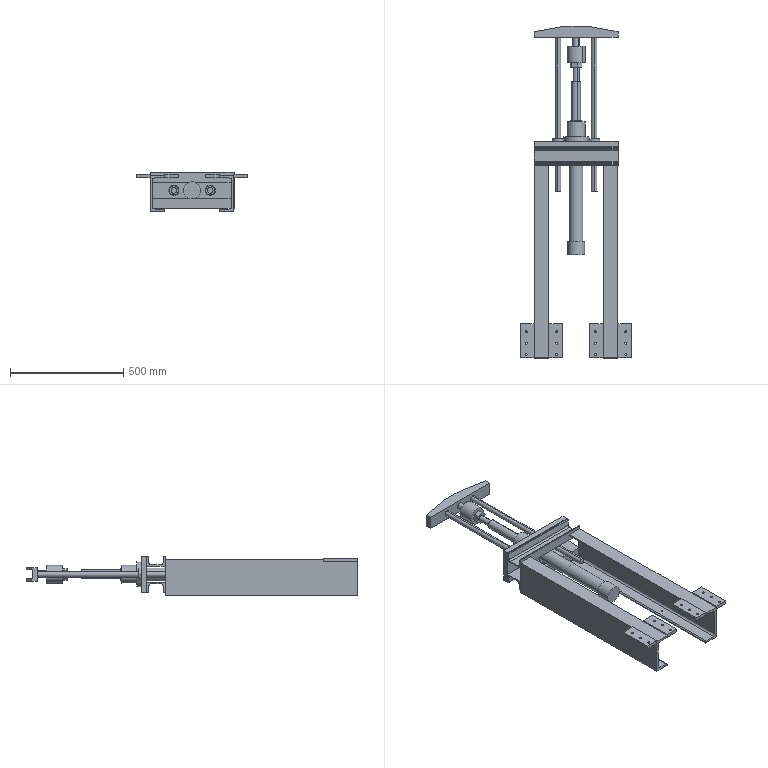Assembly | SolidWorks | mm | 17 component files | 17 solids | 221 faces | box 489.4 x 1462.46 x 173.22 mm | volume 10389265 mm3 | plane 115 | cylinder 98 | cone 8 | commonest cylinder face diameters 8.5 x16 10 x12 25 x12 40 x8 50 x8 5 x4 20 x4 60 x4
Bill of materials:
15mmSteelPlate2-331MachineTool | 2 |  | Flat rectangular plate with three round through holes in a row along its long axis; the middle hole is larger than the two end holes.
15mmSteelPlate-331MachineTool | 2 |  | Flat rectangular plate with three round through holes in a row along its length; the middle hole is larger.
BalanceCylinderBody | 1 |  | Long, slender, solid round shaft that is stepped along its axis. It has an enlarged cylindrical end section at one end, a thin raised collar near the other end, a short larger-diameter section beyond the collar, and a small step at that end's tip.
BalanceCylinderLever | 1 |  | Long, slender, solid stepped round pin: a short larger-diameter section at one end, a long middle shank, and a short reduced-diameter tip at the other end.
ChannelSteelNo.8470-2-650-331Machine | 1 |  | Short channel-section piece shown with the open side facing down (inverted U). It has one round through hole in the center of the web. The flanges taper and have rounded inner root fillets and rounded tips.
ChannelSteelNo.8470-650-331Machine | 1 |  | Straight length of channel section shown with the open side up. It has tapered flanges, rounded inner root fillets and rounded flange tips, and no holes are visible.
FloatingJointJA140-30-150 | 1 |  | Turned stepped part with a large cylindrical main body. One end has a smaller hexagonal boss with a central bore; the other end has a smaller solid cylindrical pin, coaxial with the body.
GuideRod-331 | 2 |  | Plain straight solid cylindrical rod of constant diameter with flat ends.
LinearBearingSchematic | 2 |  | Long channel section with the web vertical and the flanges pointing to one side (C-shape). The flanges taper and have rounded root fillets and tips. There is a very small dot-like mark on one flange.
NitrogenSupportChannelSteel65016a-2-331MachineTool | 1 |  | Long channel section (C-shape) with tapered flanges, rounded root fillets and rounded flange tips. No holes or other features are visible.
NitrogenSupportChannelSteel65016a-331MachineTool | 1 |  | Thin flat rectangular plate with three round through holes centered in a row along its length; the middle hole is larger than the two outer holes.
NitrogenSupportUpperPlate-331MachineTool | 1 |  | Flanged cylindrical sleeve: a hollow cylinder with a concentric through bore and a larger-diameter flange at one end.
SupportPlate-331 | 1 |  | Elongated straight bar with a C-shaped (channel-like) cross-section. Three round through holes in a row pass through the flat web: a larger hole in the middle and two smaller holes of equal size placed symmetrically on either side. Viewed from the side, the profile is symmetric: a flat raised middle section with straight tapers down toward both ends, so the flanges stand out farthest at mid-length and least at the ends.
Mates:
1. coincident | NitrogenSupportChannelSteel65016a-331MachineTool-1 face at (64.219, -126.562, 611.875) dir (0, -1, 0) | 15mmSteelPlate-331MachineTool-1 face at (82.719, -126.562, 755) dir (0, -1, 0)
2. coincident | NitrogenSupportChannelSteel65016a-331MachineTool-1 face at (82.719, -126.562, 750) dir (1, 0, 0) | 15mmSteelPlate-331MachineTool-1 face at (82.719, -126.562, 755) dir (-1, 0, 0)
3. coincident | NitrogenSupportChannelSteel65016a-331MachineTool-1 face at (17.719, -126.562, 747.35) dir (-1, 0, 0) | 15mmSteelPlate2-331MachineTool-1 face at (17.719, 23.438, 740) dir (1, 0, 0)
4. coincident | 15mmSteelPlate-331MachineTool-1 face at (82.719, -126.562, 755) dir (0, -1, 0) | 15mmSteelPlate2-331MachineTool-1 face at (-42.281, -126.562, 740) dir (0, -1, 0)
5. coincident | NitrogenSupportChannelSteel65016a-2-331MachineTool-1 face at (-286.681, -126.562, 590) dir (-1, 0, 0) | 15mmSteelPlate-331MachineTool-3 face at (-286.681, -126.562, 740) dir (1, 0, 0)
6. coincident | NitrogenSupportChannelSteel65016a-2-331MachineTool-1 face at (-268.181, -126.562, 728.125) dir (0, -1, 0) | 15mmSteelPlate-331MachineTool-3 face at (-286.681, -126.562, 740) dir (0, -1, 0)
7. coincident | NitrogenSupportChannelSteel65016a-2-331MachineTool-1 face at (-221.681, -126.562, 750) dir (1, 0, 0) | 15mmSteelPlate2-331MachineTool-2 face at (-221.681, 23.438, 755) dir (-1, 0, 0)
8. coincident | NitrogenSupportChannelSteel65016a-2-331MachineTool-1 face at (-268.181, -126.562, 728.125) dir (0, -1, 0) | 15mmSteelPlate2-331MachineTool-2 face at (-161.681, -126.562, 755) dir (0, -1, 0)
9. coincident | NitrogenSupportChannelSteel65016a-331MachineTool-1 face at (64.219, 723.438, 611.875) dir (0, 1, 0) | ChannelSteelNo.8470-650-331Machine-1 face at (83.319, 723.438, 720.223) dir (0, -1, 0)
10. coincident | NitrogenSupportUpperPlate-331MachineTool-1 face at (-96.053, 803.438, 632.765) dir (0, -1, 0) | ChannelSteelNo.8470-650-331Machine-1 face at (83.319, 803.438, 763.223) dir (0, 1, 0)
11. coincident | NitrogenSupportUpperPlate-331MachineTool-1 face at (83.319, 803.438, 604.223) dir (1, 0, 0) | ChannelSteelNo.8470-650-331Machine-1 face at (83.319, 740.578, 733.223) dir (1, 0, 0)
12. coincident | NitrogenSupportChannelSteel65016a-2-331MachineTool-1 face at (-268.181, 723.438, 728.125) dir (0, 1, 0) | ChannelSteelNo.8470-650-331Machine-1 face at (83.319, 723.438, 720.223) dir (0, -1, 0)
13. coincident | NitrogenSupportChannelSteel65016a-2-331MachineTool-1 face at (-286.681, -126.562, 590) dir (-1, 0, 0) | ChannelSteelNo.8470-650-331Machine-1 face at (-286.681, 740.578, 733.223) dir (-1, 0, 0)
14. coincident | NitrogenSupportUpperPlate-331MachineTool-1 face at (-96.053, 803.438, 632.765) dir (0, -1, 0) | ChannelSteelNo.8470-2-650-331Machine-1 face at (83.319, 803.438, 647.223) dir (0, 1, 0)
15. coincident | NitrogenSupportUpperPlate-331MachineTool-1 face at (83.319, 803.438, 604.223) dir (1, 0, 0) | ChannelSteelNo.8470-2-650-331Machine-1 face at (83.319, 786.298, 634.223) dir (1, 0, 0)
16. concentric | NitrogenSupportUpperPlate-331MachineTool-1 face at (-101.681, 828.438, 683.723) dir (0, -1, 0) r 30 | BalanceCylinderBody-1 face at (-101.681, 373.438, 683.723) dir (0, 1, 0) r 25
17. coincident | NitrogenSupportUpperPlate-331MachineTool-1 face at (-96.053, 828.438, 632.765) dir (0, 1, 0) | BalanceCylinderBody-1 face at (-46.681, 828.438, 683.723) dir (0, -1, 0)
18. concentric | BalanceCylinderBody-1 face at (-101.681, 328.438, 683.723) dir (0, -1, 0) r 39.5 | BalanceCylinderLever-1 face at (-101.681, 1090.897, 683.723) dir (0, -1, 0) r 20
19. concentric | BalanceCylinderLever-1 face at (-101.681, 1175.897, 683.723) dir (0, -1, 0) r 13.25 | FloatingJointJA140-30-150-1 face at (-101.681, 1153.897, 683.723) dir (0, -1, 0) r 39.5
20. coincident | BalanceCylinderLever-1 face at (-101.681, 1175.897, 683.723) dir (0, 1, 0) | FloatingJointJA140-30-150-1 face at (-129.34, 1175.897, 655.523) dir (0, -1, 0)
21. concentric | NitrogenSupportUpperPlate-331MachineTool-1 face at (-21.681, 828.438, 683.723) dir (0, -1, 0) r 22.5 | LinearBearingSchematic-1 face at (-21.681, 803.438, 683.723) dir (0, -1, 0) r 12.5
22. coincident | NitrogenSupportUpperPlate-331MachineTool-1 face at (-96.053, 828.438, 632.765) dir (0, 1, 0) | LinearBearingSchematic-1 face at (-41.681, 828.438, 683.723) dir (0, -1, 0)
23. concentric | NitrogenSupportUpperPlate-331MachineTool-1 face at (-181.681, 828.438, 683.723) dir (0, -1, 0) r 22.5 | LinearBearingSchematic-2 face at (-181.681, 803.438, 683.723) dir (0, -1, 0) r 20
24. coincident | LinearBearingSchematic-1 face at (-46.681, 838.438, 683.723) dir (0, 1, 0) | LinearBearingSchematic-2 face at (-206.681, 838.438, 683.723) dir (0, 1, 0)
25. concentric | FloatingJointJA140-30-150-1 face at (-101.681, 1153.897, 683.723) dir (0, -1, 0) r 15 | SupportPlate-331-1 face at (-101.681, 1285.897, 683.723) dir (0, 1, 0) r 15
26. coincident | FloatingJointJA140-30-150-1 face at (-101.681, 1305.897, 683.723) dir (0, 1, 0) | SupportPlate-331-1 face at (-286.681, 1305.897, 703.723) dir (0, 1, 0)
27. coincident | GuideRod-331-1 face at (-181.681, 1305.897, 683.723) dir (0, 1, 0) | GuideRod-331-2 face at (-21.681, 1305.897, 683.723) dir (0, 1, 0)
28. concentric | SupportPlate-331-1 face at (-21.681, 1285.897, 683.723) dir (0, 1, 0) r 12.5 | GuideRod-331-2 face at (-21.681, 1305.897, 683.723) dir (0, -1, 0) r 12.5
29. coincident | SupportPlate-331-1 face at (-286.681, 1305.897, 703.723) dir (0, 1, 0) | GuideRod-331-2 face at (-21.681, 1305.897, 683.723) dir (0, 1, 0)
30. concentric | LinearBearingSchematic-2 face at (-181.681, 803.438, 683.723) dir (0, -1, 0) r 12.5 | SupportPlate-331-1 face at (-181.681, 1285.897, 683.723) dir (0, 1, 0) r 12.5
31. concentric | LinearBearingSchematic-2 face at (-181.681, 803.438, 683.723) dir (0, -1, 0) r 12.5 | GuideRod-331-1 face at (-181.681, 1305.897, 683.723) dir (0, -1, 0) r 12.5